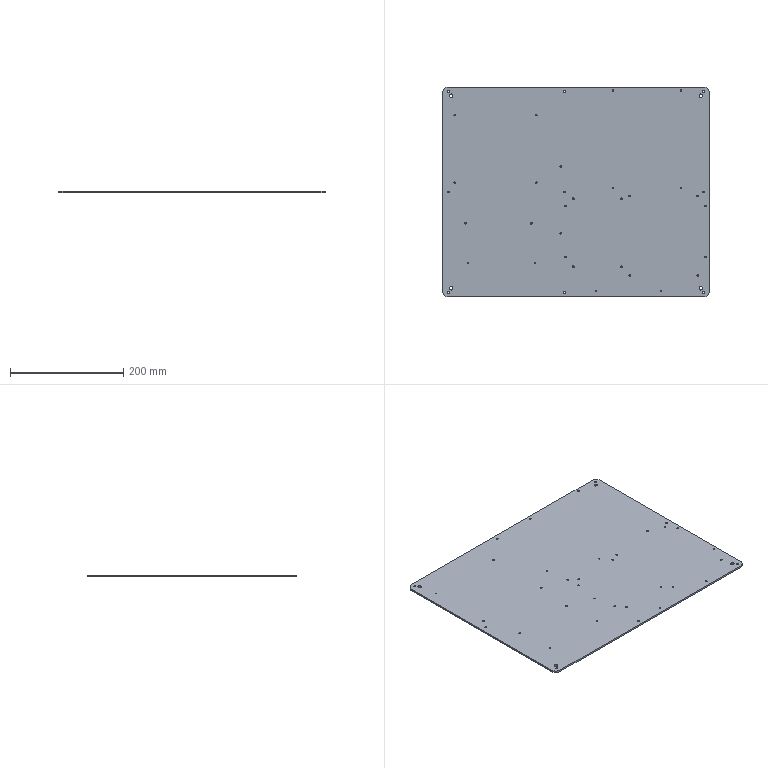CAM job | Mastercam | mm | 4 operations | part box 470 x 370 x 3
1. Contour (Ramp) | 10 - 10 平铣刀
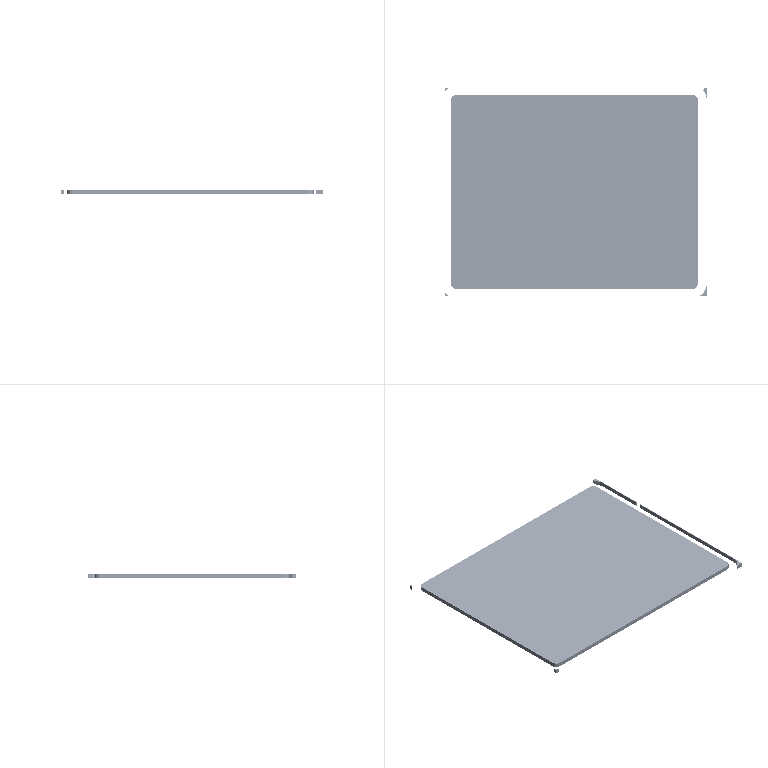2. Contour (2D) | 10 - 10 平铣刀
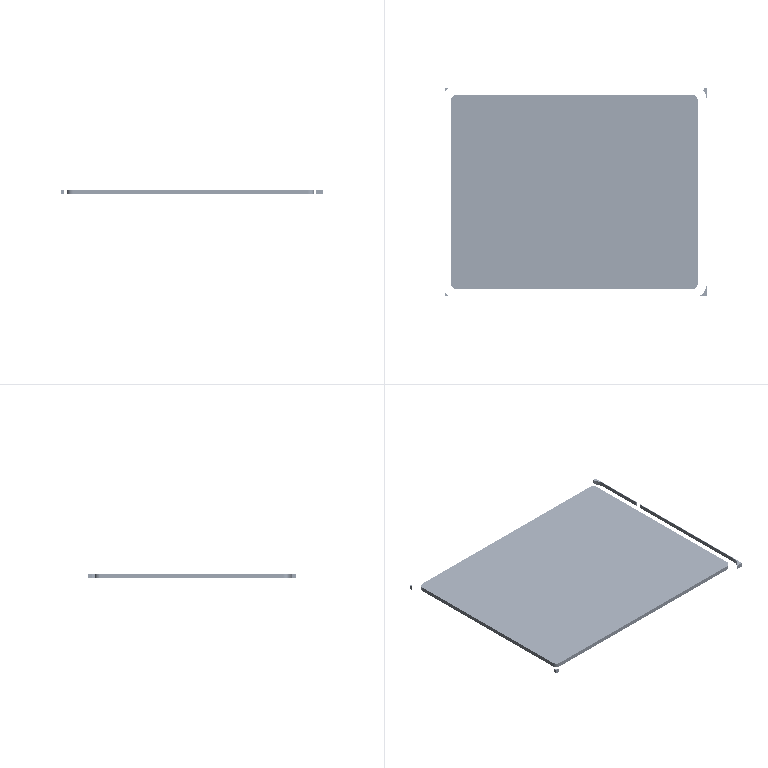3. Drill/Counterbore | 7 - 4 倒角刀
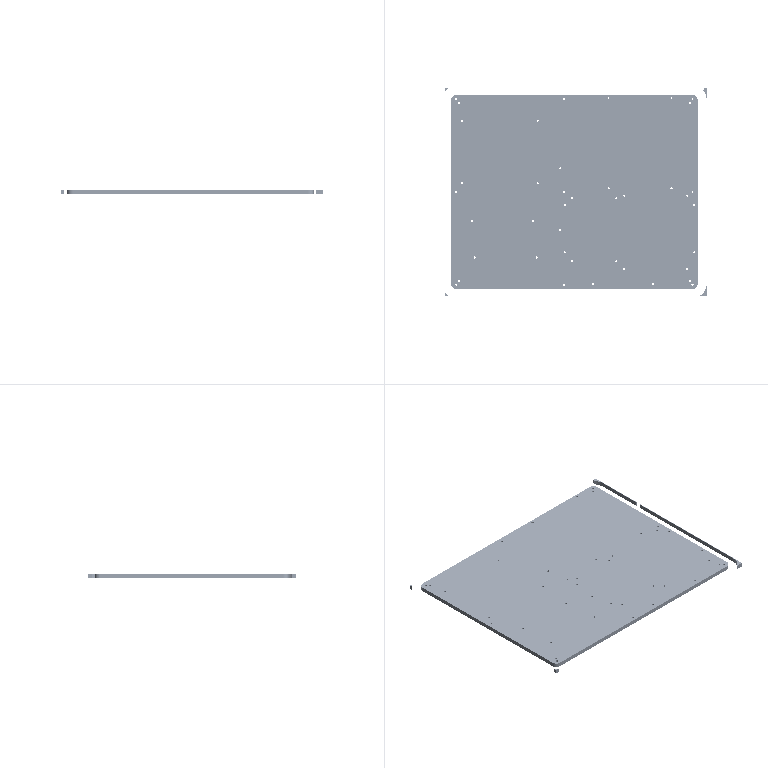4. Contour (2D chamfer) | 7 - 4 倒角刀